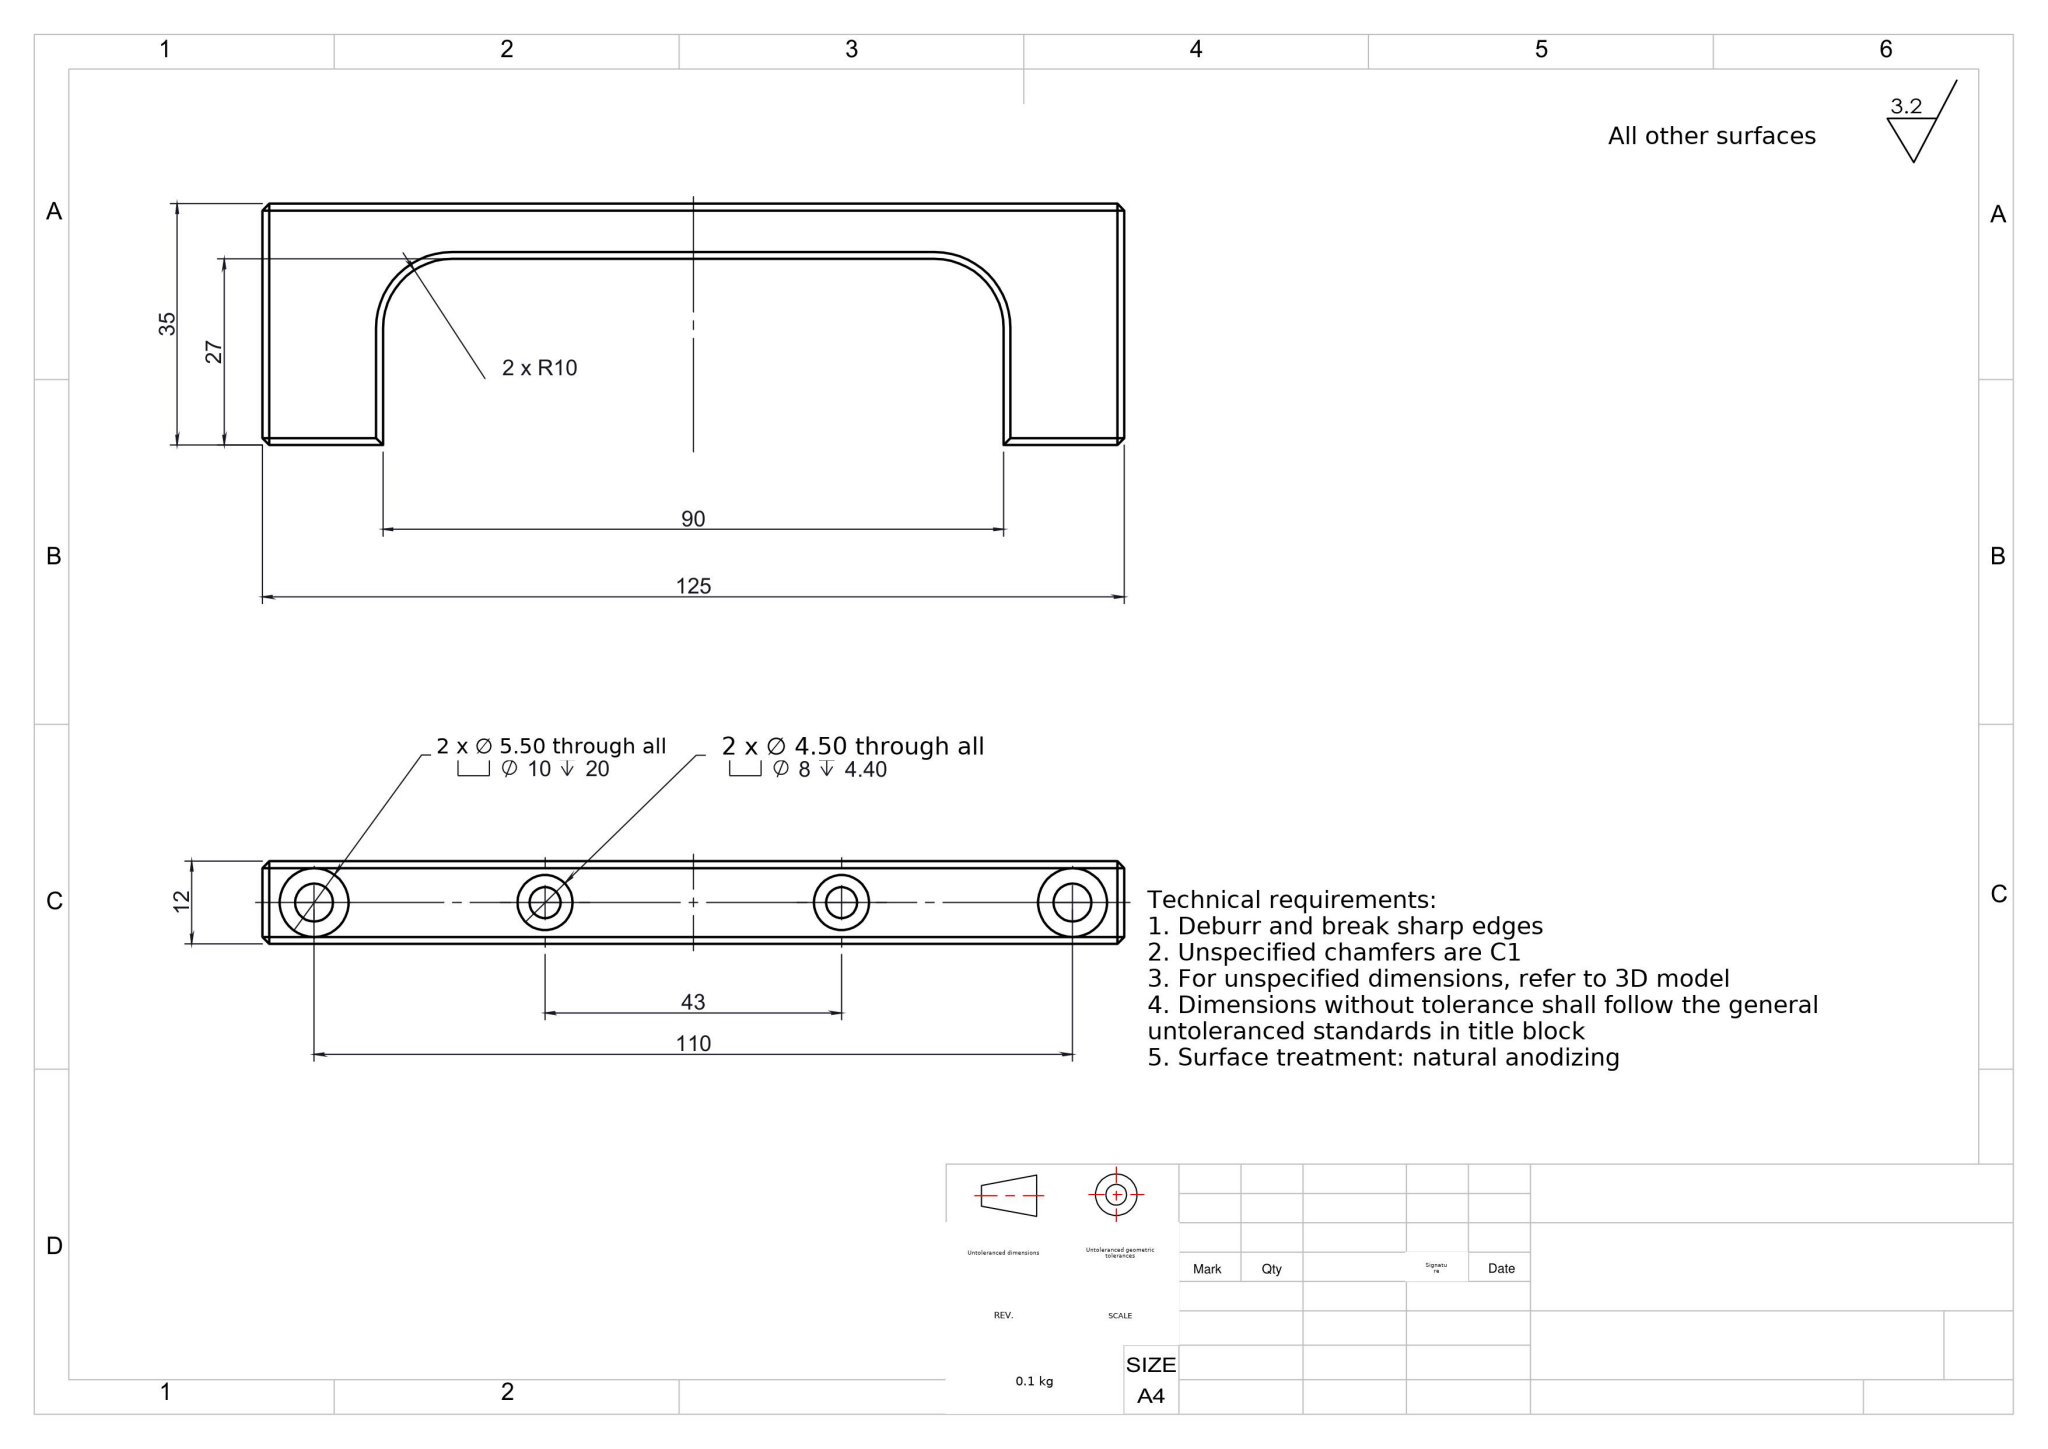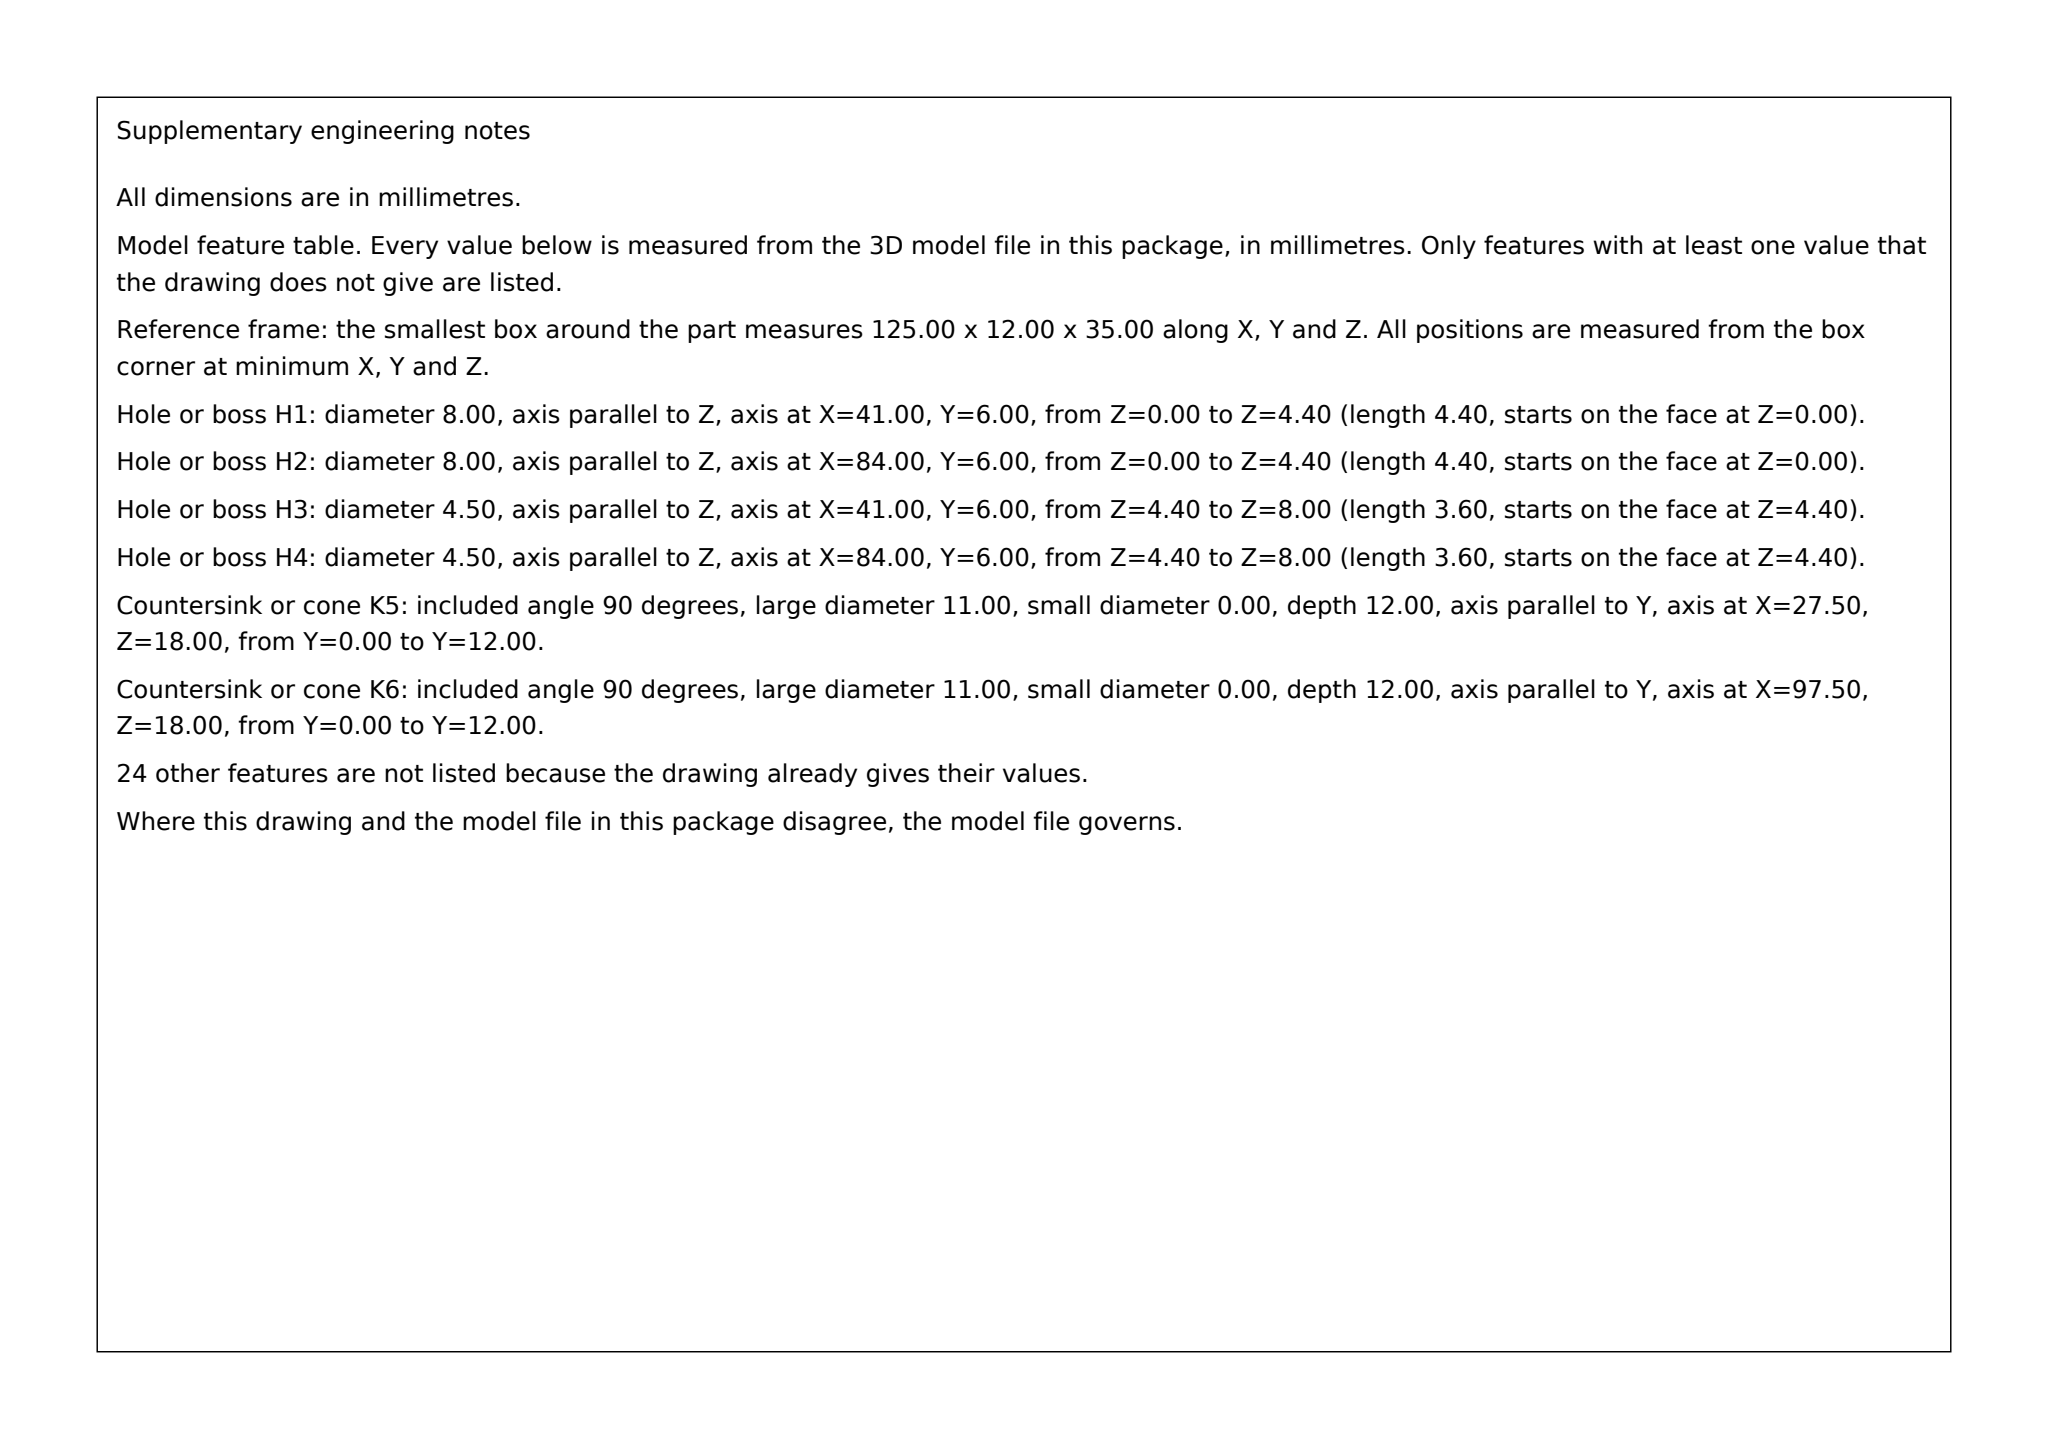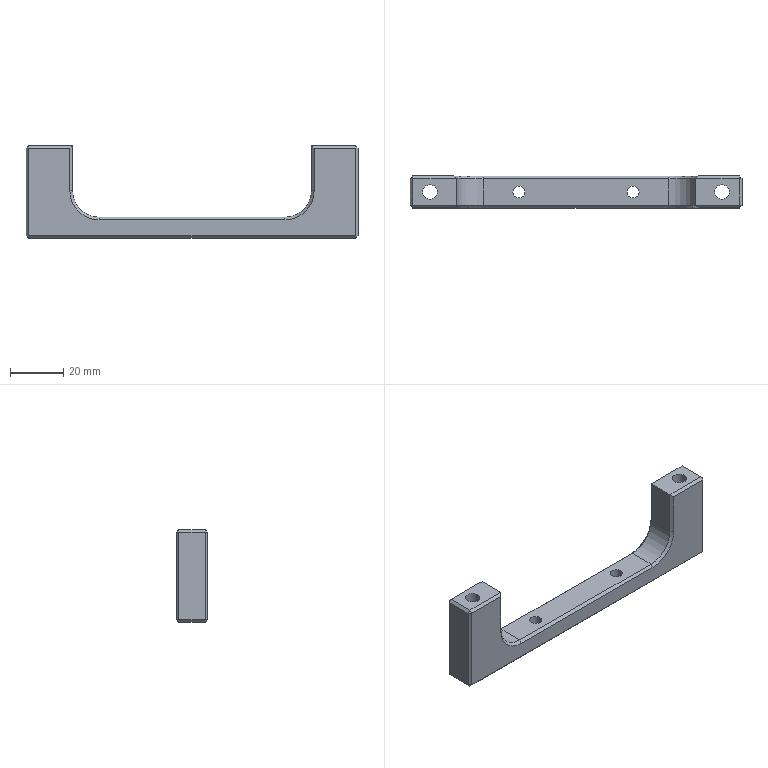Part | SolidWorks | mm | 1 solid | 66 faces | box 125 x 12 x 35 mm | volume 19060 mm3 | plane 44 | cylinder 18 | cone 4 | commonest cylinder face diameters 8 x4 4.5 x4 10 x4 5.5 x4 20 x2